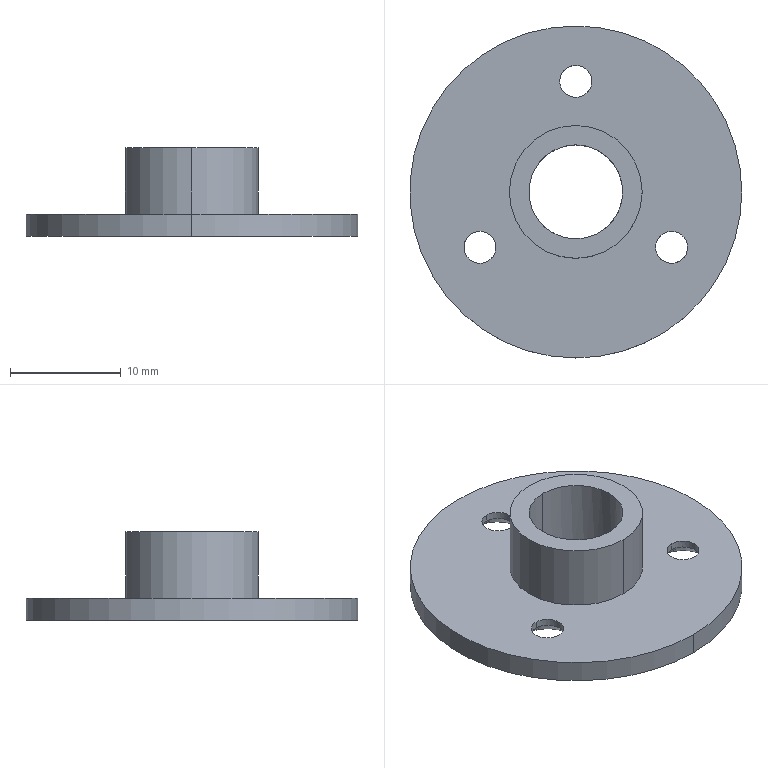CAM job | Mastercam | mm | 1 operations | part box 30 x 30 x 8
1. Drill/Counterbore | 7 - 4 倒角刀